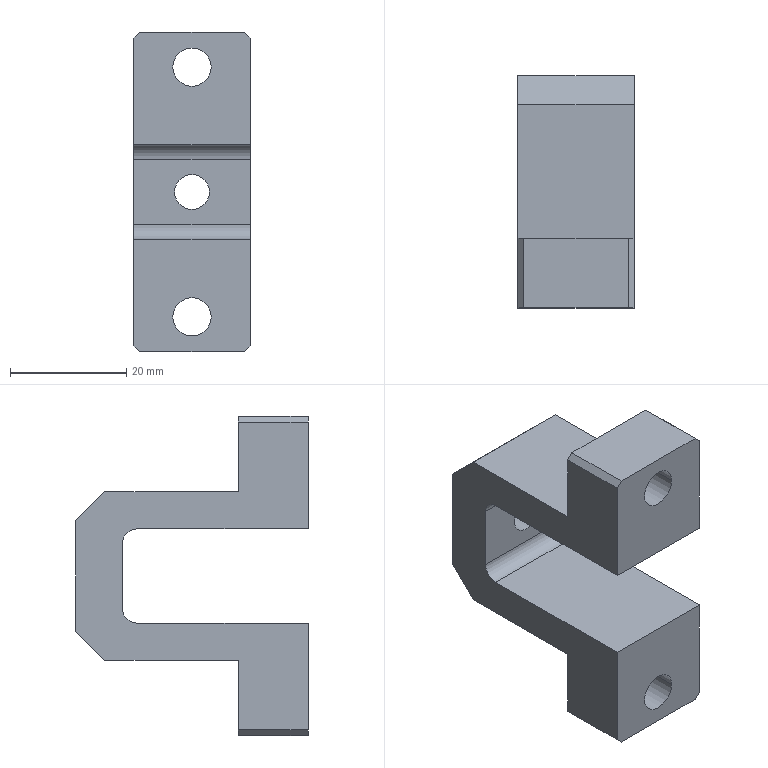Component | SolidWorks | J-TRD899MINI-2213-03PressingWheelSupport-2 | 1 solid | 28 faces | box 20 x 40 x 55 mm | volume 17554 mm3 | plane 20 | cylinder 8 | commonest cylinder face diameters 6.6 x4 6 x2 5 x2 | material 6061
build123d program:
from build123d import *

# Parameters (mm, degrees)
SKETCH1_W            = 40
SKETCH1_H            = 55
BOSS_EXTRUDE1_DEPTH  = 20
SKETCH6_W            = 28
SKETCH6_H            = 13
CUT_EXTRUDE2_DEPTH   = 40.449
CUT_EXTRUDE1_DEPTH   = 40.449
M6_CLEARANCE_HOLE1_D = 6.6
CHAMFER1_SIZE        = 5
CHAMFER2_SIZE        = 1
M6_TAPPED_HOLE1_D    = 6


with BuildPart() as part:
    # Sketch1 → Boss-Extrude1 (new body)
    with BuildSketch(Plane.XY):
        Rectangle(SKETCH1_W, SKETCH1_H)
    extrude(amount=BOSS_EXTRUDE1_DEPTH)

    # Sketch6 → Cut-Extrude2 (cut, through all)
    with BuildSketch(Plane.XY.offset(20)):
        with Locations((6, 21)):
            Rectangle(SKETCH6_W, SKETCH6_H)
        with Locations((6, -21)):
            Rectangle(SKETCH6_W, SKETCH6_H)
    extrude(amount=-CUT_EXTRUDE2_DEPTH, mode=Mode.SUBTRACT)

    # Sketch2 → Cut-Extrude1 (cut, through all)
    with BuildSketch(Plane.XY.offset(20)):
        with BuildLine():
            Line((9.5, -8.1), (-20, -8.1))
            Line((-20, -8.1), (-20, 8.1))
            Line((-20, 8.1), (9.5, 8.1))
            ThreePointArc((9.5, 8.1), (11.268, 7.368), (12, 5.6))
            Line((12, 5.6), (12, -5.6))
            ThreePointArc((12, -5.6), (11.268, -7.368), (9.5, -8.1))
        make_face()
    extrude(amount=-CUT_EXTRUDE1_DEPTH, mode=Mode.SUBTRACT)

    # M6 Clearance Hole1 (through all)
    with Locations(Plane(origin=(20, 0, 0), x_dir=(0, 0, 1), z_dir=(1, 0, 0))):
        with Locations((10, -21.5), (10, 21.5)):
            Hole(M6_CLEARANCE_HOLE1_D / 2)

    # Chamfer1
    chamfer1_edges = [part.edges().sort_by_distance(p)[0] for p in [
        (20, 14.5, 10),
        (20, -14.5, 10),
    ]]
    chamfer(chamfer1_edges, length=CHAMFER1_SIZE)

    # Chamfer2
    chamfer2_edges = [part.edges().sort_by_distance(p)[0] for p in [
        (-14, -27.5, 20),
        (-14, 27.5, 0),
        (-14, 27.5, 20),
        (-14, -27.5, 0),
    ]]
    chamfer(chamfer2_edges, length=CHAMFER2_SIZE)

    # M6 Tapped Hole1 (through all)
    with Locations(Plane(origin=(20, 0, 0), x_dir=(0, 0, -1), z_dir=(1, 0, 0))):
        with Locations((-10, 0)):
            Hole(M6_TAPPED_HOLE1_D / 2)


solid = part.part

# Placed as in the assembly
solid = solid.moved(Location((-16.663, 45.996, 191.5), (90, 90, 0)))
STEP:
#1=COLOUR_RGB('',0.7922,0.8196,0.9333);
#2=FILL_AREA_STYLE_COLOUR('',#1);
#3=FILL_AREA_STYLE('',(#2));
#4=SURFACE_STYLE_FILL_AREA(#3);
#5=SURFACE_SIDE_STYLE('',(#4));
#6=SURFACE_STYLE_USAGE(.BOTH.,#5);
#7=PRESENTATION_STYLE_ASSIGNMENT((#6));
#8=CARTESIAN_POINT('',(-0.1442,2.283,7.539));
#9=VERTEX_POINT('',#8);
#10=CARTESIAN_POINT('',(-0.3805,2.283,7.539));
#11=VERTEX_POINT('',#10);
#12=CARTESIAN_POINT('',(-0.2623,2.283,7.539));
#13=DIRECTION('',(0.,1.,0.));
#14=DIRECTION('',(0.,0.,1.));
#15=AXIS2_PLACEMENT_3D('',#12,#13,#14);
#16=CIRCLE('',#15,0.1181);
#17=EDGE_CURVE('',#9,#11,#16,.T.);
#18=ORIENTED_EDGE('',*,*,#17,.F.);
#19=CARTESIAN_POINT('',(-0.1442,2.598,7.539));
#20=VERTEX_POINT('',#19);
#21=CARTESIAN_POINT('',(-0.1442,2.598,7.539));
#22=DIRECTION('',(0.,1.,0.));
#23=VECTOR('',#22,39.37);
#24=LINE('',#21,#23);
#25=EDGE_CURVE('',#9,#20,#24,.T.);
#26=ORIENTED_EDGE('',*,*,#25,.T.);
#27=CARTESIAN_POINT('',(-0.3805,2.598,7.539));
#28=VERTEX_POINT('',#27);
#29=CARTESIAN_POINT('',(-0.2623,2.598,7.539));
#30=DIRECTION('',(0.,1.,0.));
#31=DIRECTION('',(-1.,0.,0.));
#32=AXIS2_PLACEMENT_3D('',#29,#30,#31);
#33=CIRCLE('',#32,0.1181);
#34=EDGE_CURVE('',#20,#28,#33,.T.);
#35=ORIENTED_EDGE('',*,*,#34,.T.);
#36=CARTESIAN_POINT('',(-0.3805,2.598,7.539));
#37=DIRECTION('',(0.,1.,0.));
#38=VECTOR('',#37,39.37);
#39=LINE('',#36,#38);
#40=EDGE_CURVE('',#11,#28,#39,.T.);
#41=ORIENTED_EDGE('',*,*,#40,.F.);
#42=EDGE_LOOP('',(#18,#26,#35,#41));
#43=FACE_OUTER_BOUND('',#42,.T.);
#44=CARTESIAN_POINT('',(-0.2623,2.598,7.539));
#45=DIRECTION('',(0.,1.,0.));
#46=DIRECTION('',(-1.,0.,0.));
#47=AXIS2_PLACEMENT_3D('',#44,#45,#46);
#48=CYLINDRICAL_SURFACE('',#47,0.1181);
#49=ADVANCED_FACE('',(#43),#48,.F.);
#50=CARTESIAN_POINT('',(-0.1324,1.023,8.386));
#51=VERTEX_POINT('',#50);
#52=CARTESIAN_POINT('',(-0.3923,1.023,8.386));
#53=VERTEX_POINT('',#52);
#54=CARTESIAN_POINT('',(-0.2623,1.023,8.386));
#55=DIRECTION('',(0.,1.,0.));
#56=DIRECTION('',(-1.,0.,0.));
#57=AXIS2_PLACEMENT_3D('',#54,#55,#56);
#58=CIRCLE('',#57,0.1299);
#59=EDGE_CURVE('',#51,#53,#58,.T.);
#60=ORIENTED_EDGE('',*,*,#59,.F.);
#61=CARTESIAN_POINT('',(-0.1324,1.496,8.386));
#62=VERTEX_POINT('',#61);
#63=CARTESIAN_POINT('',(-0.1324,2.598,8.386));
#64=DIRECTION('',(0.,1.,0.));
#65=VECTOR('',#64,39.37);
#66=LINE('',#63,#65);
#67=EDGE_CURVE('',#51,#62,#66,.T.);
#68=ORIENTED_EDGE('',*,*,#67,.T.);
#69=CARTESIAN_POINT('',(-0.3923,1.496,8.386));
#70=VERTEX_POINT('',#69);
#71=CARTESIAN_POINT('',(-0.2623,1.496,8.386));
#72=DIRECTION('',(0.,-1.,-0.));
#73=DIRECTION('',(0.,0.,-1.));
#74=AXIS2_PLACEMENT_3D('',#71,#72,#73);
#75=CIRCLE('',#74,0.1299);
#76=EDGE_CURVE('',#70,#62,#75,.T.);
#77=ORIENTED_EDGE('',*,*,#76,.F.);
#78=CARTESIAN_POINT('',(-0.3923,2.598,8.386));
#79=DIRECTION('',(0.,1.,0.));
#80=VECTOR('',#79,39.37);
#81=LINE('',#78,#80);
#82=EDGE_CURVE('',#53,#70,#81,.T.);
#83=ORIENTED_EDGE('',*,*,#82,.F.);
#84=EDGE_LOOP('',(#60,#68,#77,#83));
#85=FACE_OUTER_BOUND('',#84,.T.);
#86=CARTESIAN_POINT('',(-0.2623,2.598,8.386));
#87=DIRECTION('',(0.,1.,0.));
#88=DIRECTION('',(-1.,0.,0.));
#89=AXIS2_PLACEMENT_3D('',#86,#87,#88);
#90=CYLINDRICAL_SURFACE('',#89,0.1299);
#91=ADVANCED_FACE('',(#85),#90,.F.);
#92=CARTESIAN_POINT('',(-0.1324,1.023,6.693));
#93=VERTEX_POINT('',#92);
#94=CARTESIAN_POINT('',(-0.3923,1.023,6.693));
#95=VERTEX_POINT('',#94);
#96=CARTESIAN_POINT('',(-0.2623,1.023,6.693));
#97=DIRECTION('',(0.,1.,0.));
#98=DIRECTION('',(-1.,0.,0.));
#99=AXIS2_PLACEMENT_3D('',#96,#97,#98);
#100=CIRCLE('',#99,0.1299);
#101=EDGE_CURVE('',#93,#95,#100,.T.);
#102=ORIENTED_EDGE('',*,*,#101,.F.);
#103=CARTESIAN_POINT('',(-0.1324,1.496,6.693));
#104=VERTEX_POINT('',#103);
#105=CARTESIAN_POINT('',(-0.1324,2.598,6.693));
#106=DIRECTION('',(0.,1.,0.));
#107=VECTOR('',#106,39.37);
#108=LINE('',#105,#107);
#109=EDGE_CURVE('',#93,#104,#108,.T.);
#110=ORIENTED_EDGE('',*,*,#109,.T.);
#111=CARTESIAN_POINT('',(-0.3923,1.496,6.693));
#112=VERTEX_POINT('',#111);
#113=CARTESIAN_POINT('',(-0.2623,1.496,6.693));
#114=DIRECTION('',(0.,-1.,0.));
#115=DIRECTION('',(0.,0.,-1.));
#116=AXIS2_PLACEMENT_3D('',#113,#114,#115);
#117=CIRCLE('',#116,0.1299);
#118=EDGE_CURVE('',#112,#104,#117,.T.);
#119=ORIENTED_EDGE('',*,*,#118,.F.);
#120=CARTESIAN_POINT('',(-0.3923,2.598,6.693));
#121=DIRECTION('',(0.,1.,0.));
#122=VECTOR('',#121,39.37);
#123=LINE('',#120,#122);
#124=EDGE_CURVE('',#95,#112,#123,.T.);
#125=ORIENTED_EDGE('',*,*,#124,.F.);
#126=EDGE_LOOP('',(#102,#110,#119,#125));
#127=FACE_OUTER_BOUND('',#126,.T.);
#128=CARTESIAN_POINT('',(-0.2623,2.598,6.693));
#129=DIRECTION('',(0.,1.,0.));
#130=DIRECTION('',(-1.,0.,0.));
#131=AXIS2_PLACEMENT_3D('',#128,#129,#130);
#132=CYLINDRICAL_SURFACE('',#131,0.1299);
#133=ADVANCED_FACE('',(#127),#132,.F.);
#134=CARTESIAN_POINT('',(-0.2623,1.023,8.386));
#135=DIRECTION('',(0.,1.,0.));
#136=DIRECTION('',(-1.,0.,0.));
#137=AXIS2_PLACEMENT_3D('',#134,#135,#136);
#138=CIRCLE('',#137,0.1299);
#139=EDGE_CURVE('',#53,#51,#138,.T.);
#140=ORIENTED_EDGE('',*,*,#139,.T.);
#141=ORIENTED_EDGE('',*,*,#59,.T.);
#142=EDGE_LOOP('',(#140,#141));
#143=FACE_BOUND('',#142,.T.);
#144=CARTESIAN_POINT('',(0.09199,1.023,8.622));
#145=VERTEX_POINT('',#144);
#146=CARTESIAN_POINT('',(-0.6167,1.023,8.622));
#147=VERTEX_POINT('',#146);
#148=CARTESIAN_POINT('',(0.1314,1.023,8.622));
#149=DIRECTION('',(-1.,0.,0.));
#150=VECTOR('',#149,39.37);
#151=LINE('',#148,#150);
#152=EDGE_CURVE('',#145,#147,#151,.T.);
#153=ORIENTED_EDGE('',*,*,#152,.T.);
#154=CARTESIAN_POINT('',(-0.656,1.023,8.583));
#155=VERTEX_POINT('',#154);
#156=CARTESIAN_POINT('',(-0.6167,1.023,8.622));
#157=DIRECTION('',(-0.7071,0.,-0.7071));
#158=VECTOR('',#157,39.37);
#159=LINE('',#156,#158);
#160=EDGE_CURVE('',#147,#155,#159,.T.);
#161=ORIENTED_EDGE('',*,*,#160,.T.);
#162=CARTESIAN_POINT('',(-0.656,1.023,7.858));
#163=VERTEX_POINT('',#162);
#164=CARTESIAN_POINT('',(-0.656,1.023,6.457));
#165=DIRECTION('',(0.,0.,-1.));
#166=VECTOR('',#165,39.37);
#167=LINE('',#164,#166);
#168=EDGE_CURVE('',#155,#163,#167,.T.);
#169=ORIENTED_EDGE('',*,*,#168,.T.);
#170=CARTESIAN_POINT('',(0.1314,1.023,7.858));
#171=VERTEX_POINT('',#170);
#172=CARTESIAN_POINT('',(-0.656,1.023,7.858));
#173=DIRECTION('',(1.,0.,0.));
#174=VECTOR('',#173,39.37);
#175=LINE('',#172,#174);
#176=EDGE_CURVE('',#163,#171,#175,.T.);
#177=ORIENTED_EDGE('',*,*,#176,.T.);
#178=CARTESIAN_POINT('',(0.1314,1.023,8.583));
#179=VERTEX_POINT('',#178);
#180=CARTESIAN_POINT('',(0.1314,1.023,6.457));
#181=DIRECTION('',(0.,0.,-1.));
#182=VECTOR('',#181,39.37);
#183=LINE('',#180,#182);
#184=EDGE_CURVE('',#179,#171,#183,.T.);
#185=ORIENTED_EDGE('',*,*,#184,.F.);
#186=CARTESIAN_POINT('',(0.1314,1.023,8.583));
#187=DIRECTION('',(-0.7071,0.,0.7071));
#188=VECTOR('',#187,39.37);
#189=LINE('',#186,#188);
#190=EDGE_CURVE('',#179,#145,#189,.T.);
#191=ORIENTED_EDGE('',*,*,#190,.T.);
#192=EDGE_LOOP('',(#153,#161,#169,#177,#185,#191));
#193=FACE_OUTER_BOUND('',#192,.T.);
#194=CARTESIAN_POINT('',(0.1314,1.023,6.457));
#195=DIRECTION('',(0.,1.,0.));
#196=DIRECTION('',(-1.,0.,0.));
#197=AXIS2_PLACEMENT_3D('',#194,#195,#196);
#198=PLANE('',#197);
#199=ADVANCED_FACE('',(#143,#193),#198,.F.);
#200=CARTESIAN_POINT('',(-0.2623,2.598,7.539));
#201=DIRECTION('',(0.,1.,0.));
#202=DIRECTION('',(-1.,0.,0.));
#203=AXIS2_PLACEMENT_3D('',#200,#201,#202);
#204=CIRCLE('',#203,0.1181);
#205=EDGE_CURVE('',#28,#20,#204,.T.);
#206=ORIENTED_EDGE('',*,*,#205,.F.);
#207=ORIENTED_EDGE('',*,*,#34,.F.);
#208=EDGE_LOOP('',(#206,#207));
#209=FACE_BOUND('',#208,.T.);
#210=CARTESIAN_POINT('',(0.1314,2.598,7.165));
#211=VERTEX_POINT('',#210);
#212=CARTESIAN_POINT('',(0.1314,2.598,7.913));
#213=VERTEX_POINT('',#212);
#214=CARTESIAN_POINT('',(0.1314,2.598,6.457));
#215=DIRECTION('',(0.,0.,1.));
#216=VECTOR('',#215,39.37);
#217=LINE('',#214,#216);
#218=EDGE_CURVE('',#211,#213,#217,.T.);
#219=ORIENTED_EDGE('',*,*,#218,.F.);
#220=CARTESIAN_POINT('',(-0.656,2.598,7.165));
#221=VERTEX_POINT('',#220);
#222=CARTESIAN_POINT('',(0.1314,2.598,7.165));
#223=DIRECTION('',(-1.,0.,0.));
#224=VECTOR('',#223,39.37);
#225=LINE('',#222,#224);
#226=EDGE_CURVE('',#211,#221,#225,.T.);
#227=ORIENTED_EDGE('',*,*,#226,.T.);
#228=CARTESIAN_POINT('',(-0.656,2.598,7.913));
#229=VERTEX_POINT('',#228);
#230=CARTESIAN_POINT('',(-0.656,2.598,6.457));
#231=DIRECTION('',(0.,0.,1.));
#232=VECTOR('',#231,39.37);
#233=LINE('',#230,#232);
#234=EDGE_CURVE('',#221,#229,#233,.T.);
#235=ORIENTED_EDGE('',*,*,#234,.T.);
#236=CARTESIAN_POINT('',(0.1314,2.598,7.913));
#237=DIRECTION('',(1.,0.,0.));
#238=VECTOR('',#237,39.37);
#239=LINE('',#236,#238);
#240=EDGE_CURVE('',#229,#213,#239,.T.);
#241=ORIENTED_EDGE('',*,*,#240,.T.);
#242=EDGE_LOOP('',(#219,#227,#235,#241));
#243=FACE_OUTER_BOUND('',#242,.T.);
#244=CARTESIAN_POINT('',(0.1314,2.598,6.457));
#245=DIRECTION('',(0.,-1.,0.));
#246=DIRECTION('',(1.,0.,0.));
#247=AXIS2_PLACEMENT_3D('',#244,#245,#246);
#248=PLANE('',#247);
#249=ADVANCED_FACE('',(#209,#243),#248,.F.);
#250=CARTESIAN_POINT('',(-0.6167,1.496,8.622));
#251=VERTEX_POINT('',#250);
#252=CARTESIAN_POINT('',(0.09199,1.496,8.622));
#253=VERTEX_POINT('',#252);
#254=CARTESIAN_POINT('',(-0.656,1.496,8.622));
#255=DIRECTION('',(1.,0.,0.));
#256=VECTOR('',#255,39.37);
#257=LINE('',#254,#256);
#258=EDGE_CURVE('',#251,#253,#257,.T.);
#259=ORIENTED_EDGE('',*,*,#258,.F.);
#260=CARTESIAN_POINT('',(-0.6167,1.023,8.622));
#261=DIRECTION('',(0.,-1.,0.));
#262=VECTOR('',#261,39.37);
#263=LINE('',#260,#262);
#264=EDGE_CURVE('',#251,#147,#263,.T.);
#265=ORIENTED_EDGE('',*,*,#264,.T.);
#266=ORIENTED_EDGE('',*,*,#152,.F.);
#267=CARTESIAN_POINT('',(0.09199,1.023,8.622));
#268=DIRECTION('',(0.,1.,0.));
#269=VECTOR('',#268,39.37);
#270=LINE('',#267,#269);
#271=EDGE_CURVE('',#145,#253,#270,.T.);
#272=ORIENTED_EDGE('',*,*,#271,.T.);
#273=EDGE_LOOP('',(#259,#265,#266,#272));
#274=FACE_OUTER_BOUND('',#273,.T.);
#275=CARTESIAN_POINT('',(0.1314,1.023,8.622));
#276=DIRECTION('',(0.,0.,-1.));
#277=DIRECTION('',(-1.,0.,0.));
#278=AXIS2_PLACEMENT_3D('',#275,#276,#277);
#279=PLANE('',#278);
#280=ADVANCED_FACE('',(#274),#279,.F.);
#281=CARTESIAN_POINT('',(-0.2623,1.023,6.693));
#282=DIRECTION('',(0.,1.,0.));
#283=DIRECTION('',(-1.,0.,0.));
#284=AXIS2_PLACEMENT_3D('',#281,#282,#283);
#285=CIRCLE('',#284,0.1299);
#286=EDGE_CURVE('',#95,#93,#285,.T.);
#287=ORIENTED_EDGE('',*,*,#286,.T.);
#288=ORIENTED_EDGE('',*,*,#101,.T.);
#289=EDGE_LOOP('',(#287,#288));
#290=FACE_BOUND('',#289,.T.);
#291=CARTESIAN_POINT('',(0.09199,1.023,6.457));
#292=VERTEX_POINT('',#291);
#293=CARTESIAN_POINT('',(-0.6167,1.023,6.457));
#294=VERTEX_POINT('',#293);
#295=CARTESIAN_POINT('',(0.1314,1.023,6.457));
#296=DIRECTION('',(-1.,0.,0.));
#297=VECTOR('',#296,39.37);
#298=LINE('',#295,#297);
#299=EDGE_CURVE('',#292,#294,#298,.T.);
#300=ORIENTED_EDGE('',*,*,#299,.F.);
#301=CARTESIAN_POINT('',(0.1314,1.023,6.496));
#302=VERTEX_POINT('',#301);
#303=CARTESIAN_POINT('',(0.1314,1.023,6.496));
#304=DIRECTION('',(0.7071,0.,0.7071));
#305=VECTOR('',#304,39.37);
#306=LINE('',#303,#305);
#307=EDGE_CURVE('',#292,#302,#306,.T.);
#308=ORIENTED_EDGE('',*,*,#307,.T.);
#309=CARTESIAN_POINT('',(0.1314,1.023,7.22));
#310=VERTEX_POINT('',#309);
#311=CARTESIAN_POINT('',(0.1314,1.023,6.457));
#312=DIRECTION('',(0.,0.,-1.));
#313=VECTOR('',#312,39.37);
#314=LINE('',#311,#313);
#315=EDGE_CURVE('',#310,#302,#314,.T.);
#316=ORIENTED_EDGE('',*,*,#315,.F.);
#317=CARTESIAN_POINT('',(-0.656,1.023,7.22));
#318=VERTEX_POINT('',#317);
#319=CARTESIAN_POINT('',(-0.656,1.023,7.22));
#320=DIRECTION('',(1.,0.,0.));
#321=VECTOR('',#320,39.37);
#322=LINE('',#319,#321);
#323=EDGE_CURVE('',#318,#310,#322,.T.);
#324=ORIENTED_EDGE('',*,*,#323,.F.);
#325=CARTESIAN_POINT('',(-0.656,1.023,6.496));
#326=VERTEX_POINT('',#325);
#327=CARTESIAN_POINT('',(-0.656,1.023,6.457));
#328=DIRECTION('',(0.,0.,-1.));
#329=VECTOR('',#328,39.37);
#330=LINE('',#327,#329);
#331=EDGE_CURVE('',#318,#326,#330,.T.);
#332=ORIENTED_EDGE('',*,*,#331,.T.);
#333=CARTESIAN_POINT('',(-0.6167,1.023,6.457));
#334=DIRECTION('',(0.7071,0.,-0.7071));
#335=VECTOR('',#334,39.37);
#336=LINE('',#333,#335);
#337=EDGE_CURVE('',#326,#294,#336,.T.);
#338=ORIENTED_EDGE('',*,*,#337,.T.);
#339=EDGE_LOOP('',(#300,#308,#316,#324,#332,#338));
#340=FACE_OUTER_BOUND('',#339,.T.);
#341=CARTESIAN_POINT('',(0.1314,1.023,6.457));
#342=DIRECTION('',(0.,1.,0.));
#343=DIRECTION('',(-1.,0.,0.));
#344=AXIS2_PLACEMENT_3D('',#341,#342,#343);
#345=PLANE('',#344);
#346=ADVANCED_FACE('',(#290,#340),#345,.F.);
#347=CARTESIAN_POINT('',(-0.6167,1.496,6.457));
#348=VERTEX_POINT('',#347);
#349=CARTESIAN_POINT('',(0.09199,1.496,6.457));
#350=VERTEX_POINT('',#349);
#351=CARTESIAN_POINT('',(-0.656,1.496,6.457));
#352=DIRECTION('',(1.,0.,0.));
#353=VECTOR('',#352,39.37);
#354=LINE('',#351,#353);
#355=EDGE_CURVE('',#348,#350,#354,.T.);
#356=ORIENTED_EDGE('',*,*,#355,.T.);
#357=CARTESIAN_POINT('',(0.09199,1.023,6.457));
#358=DIRECTION('',(0.,-1.,0.));
#359=VECTOR('',#358,39.37);
#360=LINE('',#357,#359);
#361=EDGE_CURVE('',#350,#292,#360,.T.);
#362=ORIENTED_EDGE('',*,*,#361,.T.);
#363=ORIENTED_EDGE('',*,*,#299,.T.);
#364=CARTESIAN_POINT('',(-0.6167,1.496,6.457));
#365=DIRECTION('',(0.,1.,0.));
#366=VECTOR('',#365,39.37);
#367=LINE('',#364,#366);
#368=EDGE_CURVE('',#294,#348,#367,.T.);
#369=ORIENTED_EDGE('',*,*,#368,.T.);
#370=EDGE_LOOP('',(#356,#362,#363,#369));
#371=FACE_OUTER_BOUND('',#370,.T.);
#372=CARTESIAN_POINT('',(0.1314,1.023,6.457));
#373=DIRECTION('',(0.,0.,1.));
#374=DIRECTION('',(1.,0.,0.));
#375=AXIS2_PLACEMENT_3D('',#372,#373,#374);
#376=PLANE('',#375);
#377=ADVANCED_FACE('',(#371),#376,.F.);
#378=CARTESIAN_POINT('',(0.1314,1.496,8.583));
#379=VERTEX_POINT('',#378);
#380=CARTESIAN_POINT('',(0.1314,1.496,8.11));
#381=VERTEX_POINT('',#380);
#382=CARTESIAN_POINT('',(0.1314,1.496,8.622));
#383=DIRECTION('',(0.,0.,-1.));
#384=VECTOR('',#383,39.37);
#385=LINE('',#382,#384);
#386=EDGE_CURVE('',#379,#381,#385,.T.);
#387=ORIENTED_EDGE('',*,*,#386,.F.);
#388=CARTESIAN_POINT('',(0.1314,1.811,8.583));
#389=DIRECTION('',(0.,-1.,0.));
#390=VECTOR('',#389,39.37);
#391=LINE('',#388,#390);
#392=EDGE_CURVE('',#379,#179,#391,.T.);
#393=ORIENTED_EDGE('',*,*,#392,.T.);
#394=ORIENTED_EDGE('',*,*,#184,.T.);
#395=CARTESIAN_POINT('',(0.1314,2.185,7.858));
#396=VERTEX_POINT('',#395);
#397=CARTESIAN_POINT('',(0.1314,2.185,7.858));
#398=DIRECTION('',(0.,-1.,-0.));
#399=VECTOR('',#398,39.37);
#400=LINE('',#397,#399);
#401=EDGE_CURVE('',#396,#171,#400,.T.);
#402=ORIENTED_EDGE('',*,*,#401,.F.);
#403=CARTESIAN_POINT('',(0.1314,2.283,7.76));
#404=VERTEX_POINT('',#403);
#405=CARTESIAN_POINT('',(0.1314,2.185,7.76));
#406=DIRECTION('',(1.,0.,0.));
#407=DIRECTION('',(0.,1.,0.));
#408=AXIS2_PLACEMENT_3D('',#405,#406,#407);
#409=CIRCLE('',#408,0.09843);
#410=EDGE_CURVE('',#404,#396,#409,.T.);
#411=ORIENTED_EDGE('',*,*,#410,.F.);
#412=CARTESIAN_POINT('',(0.1314,2.283,7.319));
#413=VERTEX_POINT('',#412);
#414=CARTESIAN_POINT('',(0.1314,2.283,7.319));
#415=DIRECTION('',(0.,-0.,1.));
#416=VECTOR('',#415,39.37);
#417=LINE('',#414,#416);
#418=EDGE_CURVE('',#413,#404,#417,.T.);
#419=ORIENTED_EDGE('',*,*,#418,.F.);
#420=CARTESIAN_POINT('',(0.1314,2.185,7.22));
#421=VERTEX_POINT('',#420);
#422=CARTESIAN_POINT('',(0.1314,2.185,7.319));
#423=DIRECTION('',(1.,0.,0.));
#424=DIRECTION('',(0.,1.,0.));
#425=AXIS2_PLACEMENT_3D('',#422,#423,#424);
#426=CIRCLE('',#425,0.09843);
#427=EDGE_CURVE('',#421,#413,#426,.T.);
#428=ORIENTED_EDGE('',*,*,#427,.F.);
#429=CARTESIAN_POINT('',(0.1314,2.185,7.22));
#430=DIRECTION('',(0.,1.,0.));
#431=VECTOR('',#430,39.37);
#432=LINE('',#429,#431);
#433=EDGE_CURVE('',#310,#421,#432,.T.);
#434=ORIENTED_EDGE('',*,*,#433,.F.);
#435=ORIENTED_EDGE('',*,*,#315,.T.);
#436=CARTESIAN_POINT('',(0.1314,1.496,6.496));
#437=VERTEX_POINT('',#436);
#438=CARTESIAN_POINT('',(0.1314,1.811,6.496));
#439=DIRECTION('',(0.,1.,0.));
#440=VECTOR('',#439,39.37);
#441=LINE('',#438,#440);
#442=EDGE_CURVE('',#302,#437,#441,.T.);
#443=ORIENTED_EDGE('',*,*,#442,.T.);
#444=CARTESIAN_POINT('',(0.1314,1.496,6.969));
#445=VERTEX_POINT('',#444);
#446=CARTESIAN_POINT('',(0.1314,1.496,6.457));
#447=DIRECTION('',(0.,-0.,-1.));
#448=VECTOR('',#447,39.37);
#449=LINE('',#446,#448);
#450=EDGE_CURVE('',#445,#437,#449,.T.);
#451=ORIENTED_EDGE('',*,*,#450,.F.);
#452=CARTESIAN_POINT('',(0.1314,2.401,6.969));
#453=VERTEX_POINT('',#452);
#454=CARTESIAN_POINT('',(0.1314,2.598,6.969));
#455=DIRECTION('',(0.,-1.,0.));
#456=VECTOR('',#455,39.37);
#457=LINE('',#454,#456);
#458=EDGE_CURVE('',#453,#445,#457,.T.);
#459=ORIENTED_EDGE('',*,*,#458,.F.);
#460=CARTESIAN_POINT('',(0.1314,2.401,6.969));
#461=DIRECTION('',(0.,0.7071,0.7071));
#462=VECTOR('',#461,39.37);
#463=LINE('',#460,#462);
#464=EDGE_CURVE('',#453,#211,#463,.T.);
#465=ORIENTED_EDGE('',*,*,#464,.T.);
#466=ORIENTED_EDGE('',*,*,#218,.T.);
#467=CARTESIAN_POINT('',(0.1314,2.401,8.11));
#468=VERTEX_POINT('',#467);
#469=CARTESIAN_POINT('',(0.1314,2.598,7.913));
#470=DIRECTION('',(0.,-0.7071,0.7071));
#471=VECTOR('',#470,39.37);
#472=LINE('',#469,#471);
#473=EDGE_CURVE('',#213,#468,#472,.T.);
#474=ORIENTED_EDGE('',*,*,#473,.T.);
#475=CARTESIAN_POINT('',(0.1314,2.598,8.11));
#476=DIRECTION('',(0.,1.,0.));
#477=VECTOR('',#476,39.37);
#478=LINE('',#475,#477);
#479=EDGE_CURVE('',#381,#468,#478,.T.);
#480=ORIENTED_EDGE('',*,*,#479,.F.);
#481=EDGE_LOOP('',(#387,#393,#394,#402,#411,#419,#428,#434,#435,#443,#451,#459,#465,#466,#474,#480));
#482=FACE_OUTER_BOUND('',#481,.T.);
#483=CARTESIAN_POINT('',(0.1314,1.811,7.539));
#484=DIRECTION('',(-1.,0.,0.));
#485=DIRECTION('',(0.,-1.,0.));
#486=AXIS2_PLACEMENT_3D('',#483,#484,#485);
#487=PLANE('',#486);
#488=ADVANCED_FACE('',(#482),#487,.F.);
#489=ORIENTED_EDGE('',*,*,#168,.F.);
#490=CARTESIAN_POINT('',(-0.656,1.496,8.583));
#491=VERTEX_POINT('',#490);
#492=CARTESIAN_POINT('',(-0.656,1.496,8.583));
#493=DIRECTION('',(0.,1.,0.));
#494=VECTOR('',#493,39.37);
#495=LINE('',#492,#494);
#496=EDGE_CURVE('',#155,#491,#495,.T.);
#497=ORIENTED_EDGE('',*,*,#496,.T.);
#498=CARTESIAN_POINT('',(-0.656,1.496,8.11));
#499=VERTEX_POINT('',#498);
#500=CARTESIAN_POINT('',(-0.656,1.496,8.622));
#501=DIRECTION('',(0.,0.,-1.));
#502=VECTOR('',#501,39.37);
#503=LINE('',#500,#502);
#504=EDGE_CURVE('',#491,#499,#503,.T.);
#505=ORIENTED_EDGE('',*,*,#504,.T.);
#506=CARTESIAN_POINT('',(-0.656,2.401,8.11));
#507=VERTEX_POINT('',#506);
#508=CARTESIAN_POINT('',(-0.656,2.598,8.11));
#509=DIRECTION('',(0.,1.,0.));
#510=VECTOR('',#509,39.37);
#511=LINE('',#508,#510);
#512=EDGE_CURVE('',#499,#507,#511,.T.);
#513=ORIENTED_EDGE('',*,*,#512,.T.);
#514=CARTESIAN_POINT('',(-0.656,2.392,8.12));
#515=DIRECTION('',(0.,0.7071,-0.7071));
#516=VECTOR('',#515,39.37);
#517=LINE('',#514,#516);
#518=EDGE_CURVE('',#507,#229,#517,.T.);
#519=ORIENTED_EDGE('',*,*,#518,.T.);
#520=ORIENTED_EDGE('',*,*,#234,.F.);
#521=CARTESIAN_POINT('',(-0.656,2.401,6.969));
#522=VERTEX_POINT('',#521);
#523=CARTESIAN_POINT('',(-0.656,2.392,6.959));
#524=DIRECTION('',(0.,-0.7071,-0.7071));
#525=VECTOR('',#524,39.37);
#526=LINE('',#523,#525);
#527=EDGE_CURVE('',#221,#522,#526,.T.);
#528=ORIENTED_EDGE('',*,*,#527,.T.);
#529=CARTESIAN_POINT('',(-0.656,1.496,6.969));
#530=VERTEX_POINT('',#529);
#531=CARTESIAN_POINT('',(-0.656,2.598,6.969));
#532=DIRECTION('',(0.,-1.,0.));
#533=VECTOR('',#532,39.37);
#534=LINE('',#531,#533);
#535=EDGE_CURVE('',#522,#530,#534,.T.);
#536=ORIENTED_EDGE('',*,*,#535,.T.);
#537=CARTESIAN_POINT('',(-0.656,1.496,6.496));
#538=VERTEX_POINT('',#537);
#539=CARTESIAN_POINT('',(-0.656,1.496,6.457));
#540=DIRECTION('',(0.,-0.,-1.));
#541=VECTOR('',#540,39.37);
#542=LINE('',#539,#541);
#543=EDGE_CURVE('',#530,#538,#542,.T.);
#544=ORIENTED_EDGE('',*,*,#543,.T.);
#545=CARTESIAN_POINT('',(-0.656,1.023,6.496));
#546=DIRECTION('',(0.,-1.,0.));
#547=VECTOR('',#546,39.37);
#548=LINE('',#545,#547);
#549=EDGE_CURVE('',#538,#326,#548,.T.);
#550=ORIENTED_EDGE('',*,*,#549,.T.);
#551=ORIENTED_EDGE('',*,*,#331,.F.);
#552=CARTESIAN_POINT('',(-0.656,2.185,7.22));
#553=VERTEX_POINT('',#552);
#554=CARTESIAN_POINT('',(-0.656,2.185,7.22));
#555=DIRECTION('',(0.,1.,0.));
#556=VECTOR('',#555,39.37);
#557=LINE('',#554,#556);
#558=EDGE_CURVE('',#318,#553,#557,.T.);
#559=ORIENTED_EDGE('',*,*,#558,.T.);
#560=CARTESIAN_POINT('',(-0.656,2.283,7.319));
#561=VERTEX_POINT('',#560);
#562=CARTESIAN_POINT('',(-0.656,2.185,7.319));
#563=DIRECTION('',(1.,0.,0.));
#564=DIRECTION('',(0.,1.,0.));
#565=AXIS2_PLACEMENT_3D('',#562,#563,#564);
#566=CIRCLE('',#565,0.09843);
#567=EDGE_CURVE('',#553,#561,#566,.T.);
#568=ORIENTED_EDGE('',*,*,#567,.T.);
#569=CARTESIAN_POINT('',(-0.656,2.283,7.76));
#570=VERTEX_POINT('',#569);
#571=CARTESIAN_POINT('',(-0.656,2.283,7.319));
#572=DIRECTION('',(0.,-0.,1.));
#573=VECTOR('',#572,39.37);
#574=LINE('',#571,#573);
#575=EDGE_CURVE('',#561,#570,#574,.T.);
#576=ORIENTED_EDGE('',*,*,#575,.T.);
#577=CARTESIAN_POINT('',(-0.656,2.185,7.858));
#578=VERTEX_POINT('',#577);
#579=CARTESIAN_POINT('',(-0.656,2.185,7.76));
#580=DIRECTION('',(1.,0.,0.));
#581=DIRECTION('',(0.,1.,0.));
#582=AXIS2_PLACEMENT_3D('',#579,#580,#581);
#583=CIRCLE('',#582,0.09843);
#584=EDGE_CURVE('',#570,#578,#583,.T.);
#585=ORIENTED_EDGE('',*,*,#584,.T.);
#586=CARTESIAN_POINT('',(-0.656,2.185,7.858));
#587=DIRECTION('',(0.,-1.,-0.));
#588=VECTOR('',#587,39.37);
#589=LINE('',#586,#588);
#590=EDGE_CURVE('',#578,#163,#589,.T.);
#591=ORIENTED_EDGE('',*,*,#590,.T.);
#592=EDGE_LOOP('',(#489,#497,#505,#513,#519,#520,#528,#536,#544,#550,#551,#559,#568,#576,#585,#591));
#593=FACE_OUTER_BOUND('',#592,.T.);
#594=CARTESIAN_POINT('',(-0.656,1.811,7.539));
#595=DIRECTION('',(-1.,0.,0.));
#596=DIRECTION('',(0.,-1.,0.));
#597=AXIS2_PLACEMENT_3D('',#594,#595,#596);
#598=PLANE('',#597);
#599=ADVANCED_FACE('',(#593),#598,.T.);
#600=ORIENTED_EDGE('',*,*,#479,.T.);
#601=CARTESIAN_POINT('',(-0.656,2.401,8.11));
#602=DIRECTION('',(-1.,0.,0.));
#603=VECTOR('',#602,39.37);
#604=LINE('',#601,#603);
#605=EDGE_CURVE('',#468,#507,#604,.T.);
#606=ORIENTED_EDGE('',*,*,#605,.T.);
#607=ORIENTED_EDGE('',*,*,#512,.F.);
#608=CARTESIAN_POINT('',(-0.656,1.496,8.11));
#609=DIRECTION('',(1.,0.,0.));
#610=VECTOR('',#609,39.37);
#611=LINE('',#608,#610);
#612=EDGE_CURVE('',#499,#381,#611,.T.);
#613=ORIENTED_EDGE('',*,*,#612,.T.);
#614=EDGE_LOOP('',(#600,#606,#607,#613));
#615=FACE_OUTER_BOUND('',#614,.T.);
#616=CARTESIAN_POINT('',(-0.656,2.598,8.11));
#617=DIRECTION('',(0.,0.,-1.));
#618=DIRECTION('',(0.,1.,0.));
#619=AXIS2_PLACEMENT_3D('',#616,#617,#618);
#620=PLANE('',#619);
#621=ADVANCED_FACE('',(#615),#620,.F.);
#622=ORIENTED_EDGE('',*,*,#76,.T.);
#623=CARTESIAN_POINT('',(-0.2623,1.496,8.386));
#624=DIRECTION('',(0.,-1.,-0.));
#625=DIRECTION('',(0.,0.,-1.));
#626=AXIS2_PLACEMENT_3D('',#623,#624,#625);
#627=CIRCLE('',#626,0.1299);
#628=EDGE_CURVE('',#62,#70,#627,.T.);
#629=ORIENTED_EDGE('',*,*,#628,.T.);
#630=EDGE_LOOP('',(#622,#629));
#631=FACE_BOUND('',#630,.T.);
#632=ORIENTED_EDGE('',*,*,#504,.F.);
#633=CARTESIAN_POINT('',(-0.6167,1.496,8.622));
#634=DIRECTION('',(0.7071,-0.,0.7071));
#635=VECTOR('',#634,39.37);
#636=LINE('',#633,#635);
#637=EDGE_CURVE('',#491,#251,#636,.T.);
#638=ORIENTED_EDGE('',*,*,#637,.T.);
#639=ORIENTED_EDGE('',*,*,#258,.T.);
#640=CARTESIAN_POINT('',(0.1314,1.496,8.583));
#641=DIRECTION('',(0.7071,0.,-0.7071));
#642=VECTOR('',#641,39.37);
#643=LINE('',#640,#642);
#644=EDGE_CURVE('',#253,#379,#643,.T.);
#645=ORIENTED_EDGE('',*,*,#644,.T.);
#646=ORIENTED_EDGE('',*,*,#386,.T.);
#647=ORIENTED_EDGE('',*,*,#612,.F.);
#648=EDGE_LOOP('',(#632,#638,#639,#645,#646,#647));
#649=FACE_OUTER_BOUND('',#648,.T.);
#650=CARTESIAN_POINT('',(-0.656,1.496,8.622));
#651=DIRECTION('',(0.,-1.,-0.));
#652=DIRECTION('',(0.,0.,-1.));
#653=AXIS2_PLACEMENT_3D('',#650,#651,#652);
#654=PLANE('',#653);
#655=ADVANCED_FACE('',(#631,#649),#654,.F.);
#656=ORIENTED_EDGE('',*,*,#118,.T.);
#657=CARTESIAN_POINT('',(-0.2623,1.496,6.693));
#658=DIRECTION('',(0.,-1.,0.));
#659=DIRECTION('',(0.,0.,-1.));
#660=AXIS2_PLACEMENT_3D('',#657,#658,#659);
#661=CIRCLE('',#660,0.1299);
#662=EDGE_CURVE('',#104,#112,#661,.T.);
#663=ORIENTED_EDGE('',*,*,#662,.T.);
#664=EDGE_LOOP('',(#656,#663));
#665=FACE_BOUND('',#664,.T.);
#666=ORIENTED_EDGE('',*,*,#450,.T.);
#667=CARTESIAN_POINT('',(0.1314,1.496,6.496));
#668=DIRECTION('',(-0.7071,-0.,-0.7071));
#669=VECTOR('',#668,39.37);
#670=LINE('',#667,#669);
#671=EDGE_CURVE('',#437,#350,#670,.T.);
#672=ORIENTED_EDGE('',*,*,#671,.T.);
#673=ORIENTED_EDGE('',*,*,#355,.F.);
#674=CARTESIAN_POINT('',(-0.6167,1.496,6.457));
#675=DIRECTION('',(-0.7071,0.,0.7071));
#676=VECTOR('',#675,39.37);
#677=LINE('',#674,#676);
#678=EDGE_CURVE('',#348,#538,#677,.T.);
#679=ORIENTED_EDGE('',*,*,#678,.T.);
#680=ORIENTED_EDGE('',*,*,#543,.F.);
#681=CARTESIAN_POINT('',(-0.656,1.496,6.969));
#682=DIRECTION('',(1.,0.,0.));
#683=VECTOR('',#682,39.37);
#684=LINE('',#681,#683);
#685=EDGE_CURVE('',#530,#445,#684,.T.);
#686=ORIENTED_EDGE('',*,*,#685,.T.);
#687=EDGE_LOOP('',(#666,#672,#673,#679,#680,#686));
#688=FACE_OUTER_BOUND('',#687,.T.);
#689=CARTESIAN_POINT('',(-0.656,1.496,6.457));
#690=DIRECTION('',(0.,-1.,0.));
#691=DIRECTION('',(0.,-0.,-1.));
#692=AXIS2_PLACEMENT_3D('',#689,#690,#691);
#693=PLANE('',#692);
#694=ADVANCED_FACE('',(#665,#688),#693,.F.);
#695=ORIENTED_EDGE('',*,*,#535,.F.);
#696=CARTESIAN_POINT('',(-0.656,2.401,6.969));
#697=DIRECTION('',(1.,0.,0.));
#698=VECTOR('',#697,39.37);
#699=LINE('',#696,#698);
#700=EDGE_CURVE('',#522,#453,#699,.T.);
#701=ORIENTED_EDGE('',*,*,#700,.T.);
#702=ORIENTED_EDGE('',*,*,#458,.T.);
#703=ORIENTED_EDGE('',*,*,#685,.F.);
#704=EDGE_LOOP('',(#695,#701,#702,#703));
#705=FACE_OUTER_BOUND('',#704,.T.);
#706=CARTESIAN_POINT('',(-0.656,2.598,6.969));
#707=DIRECTION('',(0.,0.,1.));
#708=DIRECTION('',(0.,-1.,0.));
#709=AXIS2_PLACEMENT_3D('',#706,#707,#708);
#710=PLANE('',#709);
#711=ADVANCED_FACE('',(#705),#710,.F.);
#712=ORIENTED_EDGE('',*,*,#401,.T.);
#713=ORIENTED_EDGE('',*,*,#176,.F.);
#714=ORIENTED_EDGE('',*,*,#590,.F.);
#715=CARTESIAN_POINT('',(-0.656,2.185,7.858));
#716=DIRECTION('',(1.,0.,0.));
#717=VECTOR('',#716,39.37);
#718=LINE('',#715,#717);
#719=EDGE_CURVE('',#578,#396,#718,.T.);
#720=ORIENTED_EDGE('',*,*,#719,.T.);
#721=EDGE_LOOP('',(#712,#713,#714,#720));
#722=FACE_OUTER_BOUND('',#721,.T.);
#723=CARTESIAN_POINT('',(-0.656,2.185,7.858));
#724=DIRECTION('',(0.,-0.,1.));
#725=DIRECTION('',(0.,-1.,-0.));
#726=AXIS2_PLACEMENT_3D('',#723,#724,#725);
#727=PLANE('',#726);
#728=ADVANCED_FACE('',(#722),#727,.F.);
#729=ORIENTED_EDGE('',*,*,#410,.T.);
#730=ORIENTED_EDGE('',*,*,#719,.F.);
#731=ORIENTED_EDGE('',*,*,#584,.F.);
#732=CARTESIAN_POINT('',(-0.656,2.283,7.76));
#733=DIRECTION('',(1.,0.,0.));
#734=VECTOR('',#733,39.37);
#735=LINE('',#732,#734);
#736=EDGE_CURVE('',#570,#404,#735,.T.);
#737=ORIENTED_EDGE('',*,*,#736,.T.);
#738=EDGE_LOOP('',(#729,#730,#731,#737));
#739=FACE_OUTER_BOUND('',#738,.T.);
#740=CARTESIAN_POINT('',(-0.656,2.185,7.76));
#741=DIRECTION('',(1.,0.,0.));
#742=DIRECTION('',(0.,1.,0.));
#743=AXIS2_PLACEMENT_3D('',#740,#741,#742);
#744=CYLINDRICAL_SURFACE('',#743,0.09843);
#745=ADVANCED_FACE('',(#739),#744,.F.);
#746=CARTESIAN_POINT('',(-0.2623,2.283,7.539));
#747=DIRECTION('',(0.,1.,0.));
#748=DIRECTION('',(0.,0.,1.));
#749=AXIS2_PLACEMENT_3D('',#746,#747,#748);
#750=CIRCLE('',#749,0.1181);
#751=EDGE_CURVE('',#11,#9,#750,.T.);
#752=ORIENTED_EDGE('',*,*,#751,.T.);
#753=ORIENTED_EDGE('',*,*,#17,.T.);
#754=EDGE_LOOP('',(#752,#753));
#755=FACE_BOUND('',#754,.T.);
#756=ORIENTED_EDGE('',*,*,#418,.T.);
#757=ORIENTED_EDGE('',*,*,#736,.F.);
#758=ORIENTED_EDGE('',*,*,#575,.F.);
#759=CARTESIAN_POINT('',(-0.656,2.283,7.319));
#760=DIRECTION('',(1.,0.,0.));
#761=VECTOR('',#760,39.37);
#762=LINE('',#759,#761);
#763=EDGE_CURVE('',#561,#413,#762,.T.);
#764=ORIENTED_EDGE('',*,*,#763,.T.);
#765=EDGE_LOOP('',(#756,#757,#758,#764));
#766=FACE_OUTER_BOUND('',#765,.T.);
#767=CARTESIAN_POINT('',(-0.656,2.283,7.319));
#768=DIRECTION('',(0.,1.,0.));
#769=DIRECTION('',(0.,-0.,1.));
#770=AXIS2_PLACEMENT_3D('',#767,#768,#769);
#771=PLANE('',#770);
#772=ADVANCED_FACE('',(#755,#766),#771,.F.);
#773=ORIENTED_EDGE('',*,*,#427,.T.);
#774=ORIENTED_EDGE('',*,*,#763,.F.);
#775=ORIENTED_EDGE('',*,*,#567,.F.);
#776=CARTESIAN_POINT('',(-0.656,2.185,7.22));
#777=DIRECTION('',(1.,0.,0.));
#778=VECTOR('',#777,39.37);
#779=LINE('',#776,#778);
#780=EDGE_CURVE('',#553,#421,#779,.T.);
#781=ORIENTED_EDGE('',*,*,#780,.T.);
#782=EDGE_LOOP('',(#773,#774,#775,#781));
#783=FACE_OUTER_BOUND('',#782,.T.);
#784=CARTESIAN_POINT('',(-0.656,2.185,7.319));
#785=DIRECTION('',(1.,0.,0.));
#786=DIRECTION('',(0.,1.,0.));
#787=AXIS2_PLACEMENT_3D('',#784,#785,#786);
#788=CYLINDRICAL_SURFACE('',#787,0.09843);
#789=ADVANCED_FACE('',(#783),#788,.F.);
#790=ORIENTED_EDGE('',*,*,#433,.T.);
#791=ORIENTED_EDGE('',*,*,#780,.F.);
#792=ORIENTED_EDGE('',*,*,#558,.F.);
#793=ORIENTED_EDGE('',*,*,#323,.T.);
#794=EDGE_LOOP('',(#790,#791,#792,#793));
#795=FACE_OUTER_BOUND('',#794,.T.);
#796=CARTESIAN_POINT('',(-0.656,2.185,7.22));
#797=DIRECTION('',(0.,0.,-1.));
#798=DIRECTION('',(0.,1.,0.));
#799=AXIS2_PLACEMENT_3D('',#796,#797,#798);
#800=PLANE('',#799);
#801=ADVANCED_FACE('',(#795),#800,.F.);
#802=ORIENTED_EDGE('',*,*,#109,.F.);
#803=ORIENTED_EDGE('',*,*,#286,.F.);
#804=ORIENTED_EDGE('',*,*,#124,.T.);
#805=ORIENTED_EDGE('',*,*,#662,.F.);
#806=EDGE_LOOP('',(#802,#803,#804,#805));
#807=FACE_OUTER_BOUND('',#806,.T.);
#808=CARTESIAN_POINT('',(-0.2623,2.598,6.693));
#809=DIRECTION('',(0.,1.,0.));
#810=DIRECTION('',(-1.,0.,0.));
#811=AXIS2_PLACEMENT_3D('',#808,#809,#810);
#812=CYLINDRICAL_SURFACE('',#811,0.1299);
#813=ADVANCED_FACE('',(#807),#812,.F.);
#814=ORIENTED_EDGE('',*,*,#67,.F.);
#815=ORIENTED_EDGE('',*,*,#139,.F.);
#816=ORIENTED_EDGE('',*,*,#82,.T.);
#817=ORIENTED_EDGE('',*,*,#628,.F.);
#818=EDGE_LOOP('',(#814,#815,#816,#817));
#819=FACE_OUTER_BOUND('',#818,.T.);
#820=CARTESIAN_POINT('',(-0.2623,2.598,8.386));
#821=DIRECTION('',(0.,1.,0.));
#822=DIRECTION('',(-1.,0.,0.));
#823=AXIS2_PLACEMENT_3D('',#820,#821,#822);
#824=CYLINDRICAL_SURFACE('',#823,0.1299);
#825=ADVANCED_FACE('',(#819),#824,.F.);
#826=ORIENTED_EDGE('',*,*,#527,.F.);
#827=ORIENTED_EDGE('',*,*,#226,.F.);
#828=ORIENTED_EDGE('',*,*,#464,.F.);
#829=ORIENTED_EDGE('',*,*,#700,.F.);
#830=EDGE_LOOP('',(#826,#827,#828,#829));
#831=FACE_OUTER_BOUND('',#830,.T.);
#832=CARTESIAN_POINT('',(-0.656,2.401,6.969));
#833=DIRECTION('',(0.,-0.7071,0.7071));
#834=DIRECTION('',(1.,0.,0.));
#835=AXIS2_PLACEMENT_3D('',#832,#833,#834);
#836=PLANE('',#835);
#837=ADVANCED_FACE('',(#831),#836,.F.);
#838=ORIENTED_EDGE('',*,*,#518,.F.);
#839=ORIENTED_EDGE('',*,*,#605,.F.);
#840=ORIENTED_EDGE('',*,*,#473,.F.);
#841=ORIENTED_EDGE('',*,*,#240,.F.);
#842=EDGE_LOOP('',(#838,#839,#840,#841));
#843=FACE_OUTER_BOUND('',#842,.T.);
#844=CARTESIAN_POINT('',(0.1314,2.598,7.913));
#845=DIRECTION('',(0.,-0.7071,-0.7071));
#846=DIRECTION('',(1.,0.,0.));
#847=AXIS2_PLACEMENT_3D('',#844,#845,#846);
#848=PLANE('',#847);
#849=ADVANCED_FACE('',(#843),#848,.F.);
#850=ORIENTED_EDGE('',*,*,#637,.F.);
#851=ORIENTED_EDGE('',*,*,#496,.F.);
#852=ORIENTED_EDGE('',*,*,#160,.F.);
#853=ORIENTED_EDGE('',*,*,#264,.F.);
#854=EDGE_LOOP('',(#850,#851,#852,#853));
#855=FACE_OUTER_BOUND('',#854,.T.);
#856=CARTESIAN_POINT('',(-0.6167,1.023,8.622));
#857=DIRECTION('',(-0.7071,0.,0.7071));
#858=DIRECTION('',(0.,1.,0.));
#859=AXIS2_PLACEMENT_3D('',#856,#857,#858);
#860=PLANE('',#859);
#861=ADVANCED_FACE('',(#855),#860,.T.);
#862=ORIENTED_EDGE('',*,*,#644,.F.);
#863=ORIENTED_EDGE('',*,*,#271,.F.);
#864=ORIENTED_EDGE('',*,*,#190,.F.);
#865=ORIENTED_EDGE('',*,*,#392,.F.);
#866=EDGE_LOOP('',(#862,#863,#864,#865));
#867=FACE_OUTER_BOUND('',#866,.T.);
#868=CARTESIAN_POINT('',(0.1314,1.811,8.583));
#869=DIRECTION('',(-0.7071,0.,-0.7071));
#870=DIRECTION('',(0.,-1.,0.));
#871=AXIS2_PLACEMENT_3D('',#868,#869,#870);
#872=PLANE('',#871);
#873=ADVANCED_FACE('',(#867),#872,.F.);
#874=ORIENTED_EDGE('',*,*,#307,.F.);
#875=ORIENTED_EDGE('',*,*,#361,.F.);
#876=ORIENTED_EDGE('',*,*,#671,.F.);
#877=ORIENTED_EDGE('',*,*,#442,.F.);
#878=EDGE_LOOP('',(#874,#875,#876,#877));
#879=FACE_OUTER_BOUND('',#878,.T.);
#880=CARTESIAN_POINT('',(0.1314,1.811,6.496));
#881=DIRECTION('',(-0.7071,0.,0.7071));
#882=DIRECTION('',(0.,1.,0.));
#883=AXIS2_PLACEMENT_3D('',#880,#881,#882);
#884=PLANE('',#883);
#885=ADVANCED_FACE('',(#879),#884,.F.);
#886=ORIENTED_EDGE('',*,*,#337,.F.);
#887=ORIENTED_EDGE('',*,*,#549,.F.);
#888=ORIENTED_EDGE('',*,*,#678,.F.);
#889=ORIENTED_EDGE('',*,*,#368,.F.);
#890=EDGE_LOOP('',(#886,#887,#888,#889));
#891=FACE_OUTER_BOUND('',#890,.T.);
#892=CARTESIAN_POINT('',(-0.6167,1.023,6.457));
#893=DIRECTION('',(-0.7071,0.,-0.7071));
#894=DIRECTION('',(0.,-1.,0.));
#895=AXIS2_PLACEMENT_3D('',#892,#893,#894);
#896=PLANE('',#895);
#897=ADVANCED_FACE('',(#891),#896,.T.);
#898=ORIENTED_EDGE('',*,*,#25,.F.);
#899=ORIENTED_EDGE('',*,*,#751,.F.);
#900=ORIENTED_EDGE('',*,*,#40,.T.);
#901=ORIENTED_EDGE('',*,*,#205,.T.);
#902=EDGE_LOOP('',(#898,#899,#900,#901));
#903=FACE_OUTER_BOUND('',#902,.T.);
#904=CARTESIAN_POINT('',(-0.2623,2.598,7.539));
#905=DIRECTION('',(0.,1.,0.));
#906=DIRECTION('',(-1.,0.,0.));
#907=AXIS2_PLACEMENT_3D('',#904,#905,#906);
#908=CYLINDRICAL_SURFACE('',#907,0.1181);
#909=ADVANCED_FACE('',(#903),#908,.F.);
#910=CLOSED_SHELL('',(#49,#91,#133,#199,#249,#280,#346,#377,#488,#599,#621,#655,#694,#711,#728,#745,#772,#789,#801,#813,#825,#837,#849,#861,#873,#885,#897,#909));
#911=MANIFOLD_SOLID_BREP('',#910);
#912=STYLED_ITEM('',(#7),#911);
#913=PRESENTATION_LAYER_ASSIGNMENT('','',(#912));
#914=CARTESIAN_POINT('',(0.,0.,0.));
#915=DIRECTION('',(0.,0.,1.));
#916=DIRECTION('',(1.,0.,0.));
#917=AXIS2_PLACEMENT_3D('',#914,#915,#916);
#918=(LENGTH_UNIT()NAMED_UNIT(*)SI_UNIT($,.METRE.));
#919=LENGTH_MEASURE_WITH_UNIT(LENGTH_MEASURE(0.0254),#918);
#920=DIMENSIONAL_EXPONENTS(1.,0.,0.,0.,0.,0.,0.);
#921=(CONVERSION_BASED_UNIT('',#919)LENGTH_UNIT()NAMED_UNIT(#920));
#922=UNCERTAINTY_MEASURE_WITH_UNIT(LENGTH_MEASURE(0.00001),#921,'','');
#923=(NAMED_UNIT(*)PLANE_ANGLE_UNIT()SI_UNIT($,.RADIAN.));
#924=(NAMED_UNIT(*)SI_UNIT($,.STERADIAN.)SOLID_ANGLE_UNIT());
#925=(GEOMETRIC_REPRESENTATION_CONTEXT(3)GLOBAL_UNCERTAINTY_ASSIGNED_CONTEXT((#922))GLOBAL_UNIT_ASSIGNED_CONTEXT((#921,#923,#924))REPRESENTATION_CONTEXT('',''));
#926=ADVANCED_BREP_SHAPE_REPRESENTATION('',(#911,#917),#925);
#927=(LENGTH_UNIT()NAMED_UNIT(*)SI_UNIT($,.METRE.));
#928=LENGTH_MEASURE_WITH_UNIT(LENGTH_MEASURE(0.0254),#927);
#929=DIMENSIONAL_EXPONENTS(1.,0.,0.,0.,0.,0.,0.);
#930=(CONVERSION_BASED_UNIT('',#928)LENGTH_UNIT()NAMED_UNIT(#929));
#931=UNCERTAINTY_MEASURE_WITH_UNIT(LENGTH_MEASURE(0.00001),#930,'','');
#932=(NAMED_UNIT(*)PLANE_ANGLE_UNIT()SI_UNIT($,.RADIAN.));
#933=(NAMED_UNIT(*)SI_UNIT($,.STERADIAN.)SOLID_ANGLE_UNIT());
#934=(GEOMETRIC_REPRESENTATION_CONTEXT(3)GLOBAL_UNCERTAINTY_ASSIGNED_CONTEXT((#931))GLOBAL_UNIT_ASSIGNED_CONTEXT((#930,#932,#933))REPRESENTATION_CONTEXT('',''));
#935=MECHANICAL_DESIGN_GEOMETRIC_PRESENTATION_REPRESENTATION('',(#912),#934);